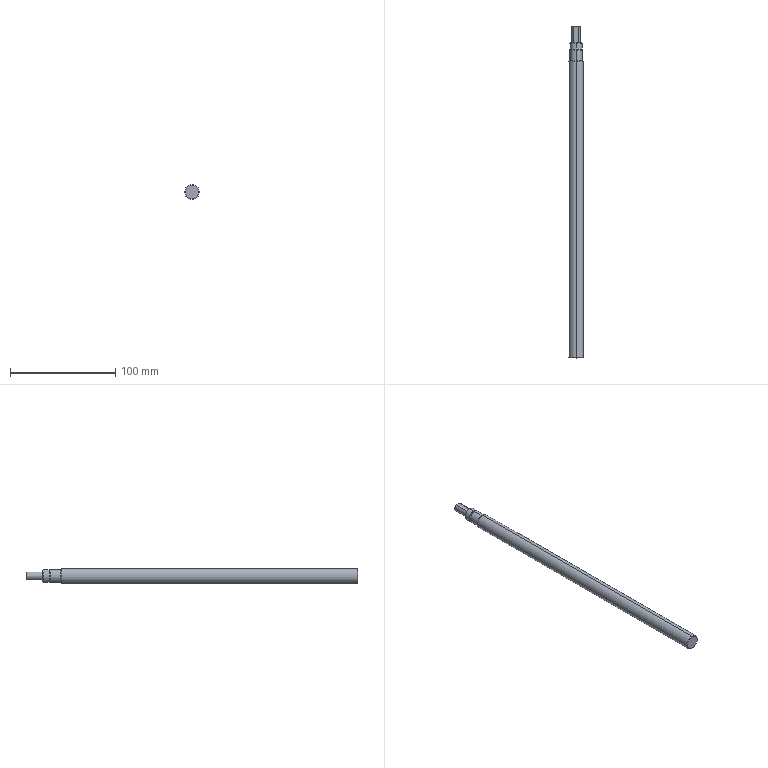Component | SolidWorks | CCDJSAdjustingScrew01-1 | 1 solid | 26 faces | box 14 x 315 x 14 mm | volume 46051 mm3 | cylinder 10 | cone 8 | plane 8 | commonest cylinder face diameters 12 x4 11.3 x2 14 x2 8 x2
build123d program:
from build123d import *

# Parameters (mm, degrees)
SKETCH2_R           = 4
BOSS_EXTRUDE1_DEPTH = 16
CHAMFER1_SIZE       = 0.5
SKETCH3_R           = 6
SKETCH3_W           = 9
SKETCH3_H           = 6.8
CUT_EXTRUDE1_DEPTH  = 16
CUT_EXTRUDE2_START  = 10
SKETCH4_OUTSIDE_W   = 79.124
SKETCH4_OUTSIDE_H   = 79.124
SKETCH4_OUTSIDE_R   = 5.65
CUT_EXTRUDE2_DEPTH  = 1.1


with BuildPart() as part:
    # Sketch1 → Revolve1 (revolve)
    with BuildSketch(Plane.XY, mode=Mode.PRIVATE) as revolve1_sk:
        Polygon((0, 0), (7, 0), (7, 282), (6, 282), (6, 299), (0, 299), align=None)
    revolve(revolve1_sk.sketch.rotate(Axis((0, 0, 0), (0, 1, 0)), 90), axis=Axis((0, 0, 0), (0, 1, 0)))

    # Sketch2 → Boss-Extrude1 (add)
    with BuildSketch(Plane(origin=(0, 299, 0), x_dir=(1, 0, 0), z_dir=(0, 1, 0))):
        with Locations(Location((0, 0, 0), (0, 0, 270))):
            Circle(SKETCH2_R)
    extrude(amount=BOSS_EXTRUDE1_DEPTH)

    # Chamfer1
    chamfer1_edges = [part.edges().sort_by_distance(p)[0] for p in [
        (0, 315, -4),
        (0, 299, 6),
        (0, 282, 7),
        (0, 0, 7),
    ]]
    chamfer(chamfer1_edges, length=CHAMFER1_SIZE)

    # Sketch3 → Cut-Extrude1 (cut)
    with BuildSketch(Plane(origin=(0, 315, 0), x_dir=(1, 0, 0), z_dir=(0, 1, 0))):
        with Locations(Location((0, 0, 0), (0, 0, 90))):
            Circle(SKETCH3_R)
        Rectangle(SKETCH3_W, SKETCH3_H, mode=Mode.SUBTRACT)
    extrude(amount=-CUT_EXTRUDE1_DEPTH, mode=Mode.SUBTRACT)

    # Sketch4 outside → Cut-Extrude2 (cut)
    with BuildSketch(Plane(origin=(0, 282, 0), x_dir=(1, 0, 0), z_dir=(0, 1, 0)).offset(CUT_EXTRUDE2_START)):
        Rectangle(SKETCH4_OUTSIDE_W, SKETCH4_OUTSIDE_H)
        with Locations(Location((0, 0, 0), (0, 0, 270))):
            Circle(SKETCH4_OUTSIDE_R, mode=Mode.SUBTRACT)
    extrude(amount=CUT_EXTRUDE2_DEPTH, mode=Mode.SUBTRACT)


solid = part.part

# Placed as in the assembly
solid = solid.moved(Location((0, 244.564, 0), (0, 0, 0)))
STEP:
#1=COLOUR_RGB('',0.7922,0.8196,0.9333);
#2=FILL_AREA_STYLE_COLOUR('',#1);
#3=FILL_AREA_STYLE('',(#2));
#4=SURFACE_STYLE_FILL_AREA(#3);
#5=SURFACE_SIDE_STYLE('',(#4));
#6=SURFACE_STYLE_USAGE(.BOTH.,#5);
#7=PRESENTATION_STYLE_ASSIGNMENT((#6));
#8=CARTESIAN_POINT('',(-0.,21.38,-0.2362));
#9=VERTEX_POINT('',#8);
#10=CARTESIAN_POINT('',(-0.,21.38,0.2362));
#11=VERTEX_POINT('',#10);
#12=CARTESIAN_POINT('',(-0.,21.38,-0.));
#13=DIRECTION('',(0.,-1.,0.));
#14=DIRECTION('',(0.,0.,1.));
#15=AXIS2_PLACEMENT_3D('',#12,#13,#14);
#16=CIRCLE('',#15,0.2362);
#17=EDGE_CURVE('',#9,#11,#16,.T.);
#18=ORIENTED_EDGE('',*,*,#17,.T.);
#19=CARTESIAN_POINT('',(-0.,21.168,0.2362));
#20=VERTEX_POINT('',#19);
#21=CARTESIAN_POINT('',(-0.,9.629,0.2362));
#22=DIRECTION('',(0.,-1.,0.));
#23=VECTOR('',#22,39.37);
#24=LINE('',#21,#23);
#25=EDGE_CURVE('',#11,#20,#24,.T.);
#26=ORIENTED_EDGE('',*,*,#25,.T.);
#27=CARTESIAN_POINT('',(-0.,21.168,-0.2362));
#28=VERTEX_POINT('',#27);
#29=CARTESIAN_POINT('',(-0.,21.168,-0.));
#30=DIRECTION('',(0.,-1.,0.));
#31=DIRECTION('',(0.,0.,1.));
#32=AXIS2_PLACEMENT_3D('',#29,#30,#31);
#33=CIRCLE('',#32,0.2362);
#34=EDGE_CURVE('',#28,#20,#33,.T.);
#35=ORIENTED_EDGE('',*,*,#34,.F.);
#36=CARTESIAN_POINT('',(-0.,9.629,-0.2362));
#37=DIRECTION('',(0.,-1.,0.));
#38=VECTOR('',#37,39.37);
#39=LINE('',#36,#38);
#40=EDGE_CURVE('',#9,#28,#39,.T.);
#41=ORIENTED_EDGE('',*,*,#40,.F.);
#42=EDGE_LOOP('',(#18,#26,#35,#41));
#43=FACE_OUTER_BOUND('',#42,.T.);
#44=CARTESIAN_POINT('',(-0.,9.629,-0.));
#45=DIRECTION('',(0.,-1.,0.));
#46=DIRECTION('',(0.,0.,-1.));
#47=AXIS2_PLACEMENT_3D('',#44,#45,#46);
#48=CYLINDRICAL_SURFACE('',#47,0.2362);
#49=ADVANCED_FACE('',(#43),#48,.T.);
#50=CARTESIAN_POINT('',(-0.,21.4,0.2165));
#51=VERTEX_POINT('',#50);
#52=CARTESIAN_POINT('',(-0.,21.4,-0.2165));
#53=VERTEX_POINT('',#52);
#54=CARTESIAN_POINT('',(-0.,21.4,-0.));
#55=DIRECTION('',(0.,1.,0.));
#56=DIRECTION('',(0.,0.,1.));
#57=AXIS2_PLACEMENT_3D('',#54,#55,#56);
#58=CIRCLE('',#57,0.2165);
#59=EDGE_CURVE('',#51,#53,#58,.T.);
#60=ORIENTED_EDGE('',*,*,#59,.F.);
#61=CARTESIAN_POINT('',(-0.,21.38,0.2362));
#62=DIRECTION('',(0.,-0.7071,0.7071));
#63=VECTOR('',#62,39.37);
#64=LINE('',#61,#63);
#65=EDGE_CURVE('',#51,#11,#64,.T.);
#66=ORIENTED_EDGE('',*,*,#65,.T.);
#67=ORIENTED_EDGE('',*,*,#17,.F.);
#68=CARTESIAN_POINT('',(-0.,21.38,-0.2362));
#69=DIRECTION('',(0.,-0.7071,-0.7071));
#70=VECTOR('',#69,39.37);
#71=LINE('',#68,#70);
#72=EDGE_CURVE('',#53,#9,#71,.T.);
#73=ORIENTED_EDGE('',*,*,#72,.F.);
#74=EDGE_LOOP('',(#60,#66,#67,#73));
#75=FACE_OUTER_BOUND('',#74,.T.);
#76=CARTESIAN_POINT('',(-0.,21.38,-0.));
#77=DIRECTION('',(0.,-1.,0.));
#78=DIRECTION('',(0.,0.,-1.));
#79=AXIS2_PLACEMENT_3D('',#76,#77,#78);
#80=CONICAL_SURFACE('',#79,0.2362,0.7854);
#81=ADVANCED_FACE('',(#75),#80,.T.);
#82=CARTESIAN_POINT('',(-0.,21.168,0.2224));
#83=VERTEX_POINT('',#82);
#84=CARTESIAN_POINT('',(-0.,21.168,-0.2224));
#85=VERTEX_POINT('',#84);
#86=CARTESIAN_POINT('',(-0.,21.168,-0.));
#87=DIRECTION('',(0.,1.,0.));
#88=DIRECTION('',(0.,0.,1.));
#89=AXIS2_PLACEMENT_3D('',#86,#87,#88);
#90=CIRCLE('',#89,0.2224);
#91=EDGE_CURVE('',#83,#85,#90,.T.);
#92=ORIENTED_EDGE('',*,*,#91,.F.);
#93=CARTESIAN_POINT('',(-0.,21.125,0.2224));
#94=VERTEX_POINT('',#93);
#95=CARTESIAN_POINT('',(-0.,21.168,0.2224));
#96=DIRECTION('',(0.,-1.,0.));
#97=VECTOR('',#96,39.37);
#98=LINE('',#95,#97);
#99=EDGE_CURVE('',#83,#94,#98,.T.);
#100=ORIENTED_EDGE('',*,*,#99,.T.);
#101=CARTESIAN_POINT('',(-0.,21.125,-0.2224));
#102=VERTEX_POINT('',#101);
#103=CARTESIAN_POINT('',(-0.,21.125,-0.));
#104=DIRECTION('',(0.,1.,0.));
#105=DIRECTION('',(0.,0.,1.));
#106=AXIS2_PLACEMENT_3D('',#103,#104,#105);
#107=CIRCLE('',#106,0.2224);
#108=EDGE_CURVE('',#94,#102,#107,.T.);
#109=ORIENTED_EDGE('',*,*,#108,.T.);
#110=CARTESIAN_POINT('',(-0.,21.168,-0.2224));
#111=DIRECTION('',(0.,-1.,0.));
#112=VECTOR('',#111,39.37);
#113=LINE('',#110,#112);
#114=EDGE_CURVE('',#85,#102,#113,.T.);
#115=ORIENTED_EDGE('',*,*,#114,.F.);
#116=EDGE_LOOP('',(#92,#100,#109,#115));
#117=FACE_OUTER_BOUND('',#116,.T.);
#118=CARTESIAN_POINT('',(-0.,21.168,-0.));
#119=DIRECTION('',(0.,-1.,0.));
#120=DIRECTION('',(0.,0.,-1.));
#121=AXIS2_PLACEMENT_3D('',#118,#119,#120);
#122=CYLINDRICAL_SURFACE('',#121,0.2224);
#123=ADVANCED_FACE('',(#117),#122,.T.);
#124=CARTESIAN_POINT('',(-0.,20.731,0.2559));
#125=VERTEX_POINT('',#124);
#126=CARTESIAN_POINT('',(-0.,20.731,-0.2559));
#127=VERTEX_POINT('',#126);
#128=CARTESIAN_POINT('',(-0.,20.731,-0.));
#129=DIRECTION('',(0.,1.,0.));
#130=DIRECTION('',(0.,0.,1.));
#131=AXIS2_PLACEMENT_3D('',#128,#129,#130);
#132=CIRCLE('',#131,0.2559);
#133=EDGE_CURVE('',#125,#127,#132,.T.);
#134=ORIENTED_EDGE('',*,*,#133,.F.);
#135=CARTESIAN_POINT('',(-0.,20.711,0.2756));
#136=VERTEX_POINT('',#135);
#137=CARTESIAN_POINT('',(-0.,20.711,0.2756));
#138=DIRECTION('',(0.,-0.7071,0.7071));
#139=VECTOR('',#138,39.37);
#140=LINE('',#137,#139);
#141=EDGE_CURVE('',#125,#136,#140,.T.);
#142=ORIENTED_EDGE('',*,*,#141,.T.);
#143=CARTESIAN_POINT('',(-0.,20.711,-0.2756));
#144=VERTEX_POINT('',#143);
#145=CARTESIAN_POINT('',(-0.,20.711,-0.));
#146=DIRECTION('',(0.,-1.,0.));
#147=DIRECTION('',(0.,0.,1.));
#148=AXIS2_PLACEMENT_3D('',#145,#146,#147);
#149=CIRCLE('',#148,0.2756);
#150=EDGE_CURVE('',#144,#136,#149,.T.);
#151=ORIENTED_EDGE('',*,*,#150,.F.);
#152=CARTESIAN_POINT('',(-0.,20.711,-0.2756));
#153=DIRECTION('',(0.,-0.7071,-0.7071));
#154=VECTOR('',#153,39.37);
#155=LINE('',#152,#154);
#156=EDGE_CURVE('',#127,#144,#155,.T.);
#157=ORIENTED_EDGE('',*,*,#156,.F.);
#158=EDGE_LOOP('',(#134,#142,#151,#157));
#159=FACE_OUTER_BOUND('',#158,.T.);
#160=CARTESIAN_POINT('',(-0.,20.711,-0.));
#161=DIRECTION('',(0.,-1.,0.));
#162=DIRECTION('',(0.,0.,-1.));
#163=AXIS2_PLACEMENT_3D('',#160,#161,#162);
#164=CONICAL_SURFACE('',#163,0.2756,0.7854);
#165=ADVANCED_FACE('',(#159),#164,.T.);
#166=CARTESIAN_POINT('',(-0.,9.629,-0.2559));
#167=VERTEX_POINT('',#166);
#168=CARTESIAN_POINT('',(-0.,9.629,0.2559));
#169=VERTEX_POINT('',#168);
#170=CARTESIAN_POINT('',(-0.,9.629,-0.));
#171=DIRECTION('',(0.,-1.,0.));
#172=DIRECTION('',(0.,0.,-1.));
#173=AXIS2_PLACEMENT_3D('',#170,#171,#172);
#174=CIRCLE('',#173,0.2559);
#175=EDGE_CURVE('',#167,#169,#174,.T.);
#176=ORIENTED_EDGE('',*,*,#175,.F.);
#177=CARTESIAN_POINT('',(-0.,9.648,-0.2756));
#178=VERTEX_POINT('',#177);
#179=CARTESIAN_POINT('',(-0.,9.629,-0.2559));
#180=DIRECTION('',(0.,0.7071,-0.7071));
#181=VECTOR('',#180,39.37);
#182=LINE('',#179,#181);
#183=EDGE_CURVE('',#167,#178,#182,.T.);
#184=ORIENTED_EDGE('',*,*,#183,.T.);
#185=CARTESIAN_POINT('',(-0.,9.648,0.2756));
#186=VERTEX_POINT('',#185);
#187=CARTESIAN_POINT('',(-0.,9.648,-0.));
#188=DIRECTION('',(0.,1.,0.));
#189=DIRECTION('',(0.,0.,-1.));
#190=AXIS2_PLACEMENT_3D('',#187,#188,#189);
#191=CIRCLE('',#190,0.2756);
#192=EDGE_CURVE('',#186,#178,#191,.T.);
#193=ORIENTED_EDGE('',*,*,#192,.F.);
#194=CARTESIAN_POINT('',(-0.,9.629,0.2559));
#195=DIRECTION('',(0.,0.7071,0.7071));
#196=VECTOR('',#195,39.37);
#197=LINE('',#194,#196);
#198=EDGE_CURVE('',#169,#186,#197,.T.);
#199=ORIENTED_EDGE('',*,*,#198,.F.);
#200=EDGE_LOOP('',(#176,#184,#193,#199));
#201=FACE_OUTER_BOUND('',#200,.T.);
#202=CARTESIAN_POINT('',(-0.,9.629,-0.));
#203=DIRECTION('',(0.,1.,0.));
#204=DIRECTION('',(0.,0.,1.));
#205=AXIS2_PLACEMENT_3D('',#202,#203,#204);
#206=CONICAL_SURFACE('',#205,0.2559,0.7854);
#207=ADVANCED_FACE('',(#201),#206,.T.);
#208=ORIENTED_EDGE('',*,*,#150,.T.);
#209=CARTESIAN_POINT('',(-0.,9.629,0.2756));
#210=DIRECTION('',(0.,-1.,0.));
#211=VECTOR('',#210,39.37);
#212=LINE('',#209,#211);
#213=EDGE_CURVE('',#136,#186,#212,.T.);
#214=ORIENTED_EDGE('',*,*,#213,.T.);
#215=ORIENTED_EDGE('',*,*,#192,.T.);
#216=CARTESIAN_POINT('',(-0.,9.629,-0.2756));
#217=DIRECTION('',(0.,-1.,0.));
#218=VECTOR('',#217,39.37);
#219=LINE('',#216,#218);
#220=EDGE_CURVE('',#144,#178,#219,.T.);
#221=ORIENTED_EDGE('',*,*,#220,.F.);
#222=EDGE_LOOP('',(#208,#214,#215,#221));
#223=FACE_OUTER_BOUND('',#222,.T.);
#224=CARTESIAN_POINT('',(-0.,9.629,-0.));
#225=DIRECTION('',(0.,-1.,0.));
#226=DIRECTION('',(0.,0.,-1.));
#227=AXIS2_PLACEMENT_3D('',#224,#225,#226);
#228=CYLINDRICAL_SURFACE('',#227,0.2756);
#229=ADVANCED_FACE('',(#223),#228,.T.);
#230=CARTESIAN_POINT('',(-0.,21.125,-0.2362));
#231=VERTEX_POINT('',#230);
#232=CARTESIAN_POINT('',(-0.,21.125,0.2362));
#233=VERTEX_POINT('',#232);
#234=CARTESIAN_POINT('',(-0.,21.125,-0.));
#235=DIRECTION('',(0.,-1.,0.));
#236=DIRECTION('',(0.,0.,1.));
#237=AXIS2_PLACEMENT_3D('',#234,#235,#236);
#238=CIRCLE('',#237,0.2362);
#239=EDGE_CURVE('',#231,#233,#238,.T.);
#240=ORIENTED_EDGE('',*,*,#239,.T.);
#241=CARTESIAN_POINT('',(-0.,20.731,0.2362));
#242=VERTEX_POINT('',#241);
#243=CARTESIAN_POINT('',(-0.,9.629,0.2362));
#244=DIRECTION('',(0.,-1.,0.));
#245=VECTOR('',#244,39.37);
#246=LINE('',#243,#245);
#247=EDGE_CURVE('',#233,#242,#246,.T.);
#248=ORIENTED_EDGE('',*,*,#247,.T.);
#249=CARTESIAN_POINT('',(-0.,20.731,-0.2362));
#250=VERTEX_POINT('',#249);
#251=CARTESIAN_POINT('',(-0.,20.731,-0.));
#252=DIRECTION('',(0.,-1.,0.));
#253=DIRECTION('',(0.,0.,-1.));
#254=AXIS2_PLACEMENT_3D('',#251,#252,#253);
#255=CIRCLE('',#254,0.2362);
#256=EDGE_CURVE('',#250,#242,#255,.T.);
#257=ORIENTED_EDGE('',*,*,#256,.F.);
#258=CARTESIAN_POINT('',(-0.,9.629,-0.2362));
#259=DIRECTION('',(0.,-1.,0.));
#260=VECTOR('',#259,39.37);
#261=LINE('',#258,#260);
#262=EDGE_CURVE('',#231,#250,#261,.T.);
#263=ORIENTED_EDGE('',*,*,#262,.F.);
#264=EDGE_LOOP('',(#240,#248,#257,#263));
#265=FACE_OUTER_BOUND('',#264,.T.);
#266=CARTESIAN_POINT('',(-0.,9.629,-0.));
#267=DIRECTION('',(0.,-1.,0.));
#268=DIRECTION('',(0.,0.,-1.));
#269=AXIS2_PLACEMENT_3D('',#266,#267,#268);
#270=CYLINDRICAL_SURFACE('',#269,0.2362);
#271=ADVANCED_FACE('',(#265),#270,.T.);
#272=ORIENTED_EDGE('',*,*,#247,.F.);
#273=CARTESIAN_POINT('',(-0.,21.125,-0.));
#274=DIRECTION('',(0.,-1.,0.));
#275=DIRECTION('',(0.,0.,1.));
#276=AXIS2_PLACEMENT_3D('',#273,#274,#275);
#277=CIRCLE('',#276,0.2362);
#278=EDGE_CURVE('',#233,#231,#277,.T.);
#279=ORIENTED_EDGE('',*,*,#278,.T.);
#280=ORIENTED_EDGE('',*,*,#262,.T.);
#281=CARTESIAN_POINT('',(-0.,20.731,-0.));
#282=DIRECTION('',(0.,-1.,0.));
#283=DIRECTION('',(0.,0.,-1.));
#284=AXIS2_PLACEMENT_3D('',#281,#282,#283);
#285=CIRCLE('',#284,0.2362);
#286=EDGE_CURVE('',#242,#250,#285,.T.);
#287=ORIENTED_EDGE('',*,*,#286,.F.);
#288=EDGE_LOOP('',(#272,#279,#280,#287));
#289=FACE_OUTER_BOUND('',#288,.T.);
#290=CARTESIAN_POINT('',(-0.,9.629,-0.));
#291=DIRECTION('',(0.,-1.,0.));
#292=DIRECTION('',(0.,0.,-1.));
#293=AXIS2_PLACEMENT_3D('',#290,#291,#292);
#294=CYLINDRICAL_SURFACE('',#293,0.2362);
#295=ADVANCED_FACE('',(#289),#294,.T.);
#296=CARTESIAN_POINT('',(-0.,9.629,-0.));
#297=DIRECTION('',(0.,-1.,0.));
#298=DIRECTION('',(0.,0.,-1.));
#299=AXIS2_PLACEMENT_3D('',#296,#297,#298);
#300=CIRCLE('',#299,0.2559);
#301=EDGE_CURVE('',#169,#167,#300,.T.);
#302=ORIENTED_EDGE('',*,*,#301,.T.);
#303=ORIENTED_EDGE('',*,*,#175,.T.);
#304=EDGE_LOOP('',(#302,#303));
#305=FACE_OUTER_BOUND('',#304,.T.);
#306=CARTESIAN_POINT('',(-0.,9.629,-0.));
#307=DIRECTION('',(0.,-1.,0.));
#308=DIRECTION('',(0.,0.,-1.));
#309=AXIS2_PLACEMENT_3D('',#306,#307,#308);
#310=PLANE('',#309);
#311=ADVANCED_FACE('',(#305),#310,.T.);
#312=ORIENTED_EDGE('',*,*,#213,.F.);
#313=CARTESIAN_POINT('',(-0.,20.711,-0.));
#314=DIRECTION('',(0.,-1.,0.));
#315=DIRECTION('',(0.,0.,1.));
#316=AXIS2_PLACEMENT_3D('',#313,#314,#315);
#317=CIRCLE('',#316,0.2756);
#318=EDGE_CURVE('',#136,#144,#317,.T.);
#319=ORIENTED_EDGE('',*,*,#318,.T.);
#320=ORIENTED_EDGE('',*,*,#220,.T.);
#321=CARTESIAN_POINT('',(-0.,9.648,-0.));
#322=DIRECTION('',(0.,1.,0.));
#323=DIRECTION('',(0.,0.,-1.));
#324=AXIS2_PLACEMENT_3D('',#321,#322,#323);
#325=CIRCLE('',#324,0.2756);
#326=EDGE_CURVE('',#178,#186,#325,.T.);
#327=ORIENTED_EDGE('',*,*,#326,.T.);
#328=EDGE_LOOP('',(#312,#319,#320,#327));
#329=FACE_OUTER_BOUND('',#328,.T.);
#330=CARTESIAN_POINT('',(-0.,9.629,-0.));
#331=DIRECTION('',(0.,-1.,0.));
#332=DIRECTION('',(0.,0.,-1.));
#333=AXIS2_PLACEMENT_3D('',#330,#331,#332);
#334=CYLINDRICAL_SURFACE('',#333,0.2756);
#335=ADVANCED_FACE('',(#329),#334,.T.);
#336=CARTESIAN_POINT('',(-0.,20.731,-0.));
#337=DIRECTION('',(0.,1.,0.));
#338=DIRECTION('',(0.,0.,1.));
#339=AXIS2_PLACEMENT_3D('',#336,#337,#338);
#340=CIRCLE('',#339,0.2559);
#341=EDGE_CURVE('',#127,#125,#340,.T.);
#342=ORIENTED_EDGE('',*,*,#341,.T.);
#343=ORIENTED_EDGE('',*,*,#133,.T.);
#344=EDGE_LOOP('',(#342,#343));
#345=FACE_OUTER_BOUND('',#344,.T.);
#346=ORIENTED_EDGE('',*,*,#256,.T.);
#347=ORIENTED_EDGE('',*,*,#286,.T.);
#348=EDGE_LOOP('',(#346,#347));
#349=FACE_BOUND('',#348,.T.);
#350=CARTESIAN_POINT('',(0.2756,20.731,-0.));
#351=DIRECTION('',(0.,1.,0.));
#352=DIRECTION('',(0.,0.,1.));
#353=AXIS2_PLACEMENT_3D('',#350,#351,#352);
#354=PLANE('',#353);
#355=ADVANCED_FACE('',(#345,#349),#354,.T.);
#356=ORIENTED_EDGE('',*,*,#183,.F.);
#357=ORIENTED_EDGE('',*,*,#301,.F.);
#358=ORIENTED_EDGE('',*,*,#198,.T.);
#359=ORIENTED_EDGE('',*,*,#326,.F.);
#360=EDGE_LOOP('',(#356,#357,#358,#359));
#361=FACE_OUTER_BOUND('',#360,.T.);
#362=CARTESIAN_POINT('',(-0.,9.629,-0.));
#363=DIRECTION('',(0.,1.,0.));
#364=DIRECTION('',(0.,0.,1.));
#365=AXIS2_PLACEMENT_3D('',#362,#363,#364);
#366=CONICAL_SURFACE('',#365,0.2559,0.7854);
#367=ADVANCED_FACE('',(#361),#366,.T.);
#368=ORIENTED_EDGE('',*,*,#141,.F.);
#369=ORIENTED_EDGE('',*,*,#341,.F.);
#370=ORIENTED_EDGE('',*,*,#156,.T.);
#371=ORIENTED_EDGE('',*,*,#318,.F.);
#372=EDGE_LOOP('',(#368,#369,#370,#371));
#373=FACE_OUTER_BOUND('',#372,.T.);
#374=CARTESIAN_POINT('',(-0.,20.711,-0.));
#375=DIRECTION('',(0.,-1.,0.));
#376=DIRECTION('',(0.,0.,-1.));
#377=AXIS2_PLACEMENT_3D('',#374,#375,#376);
#378=CONICAL_SURFACE('',#377,0.2756,0.7854);
#379=ADVANCED_FACE('',(#373),#378,.T.);
#380=ORIENTED_EDGE('',*,*,#34,.T.);
#381=CARTESIAN_POINT('',(-0.,21.168,-0.));
#382=DIRECTION('',(0.,-1.,0.));
#383=DIRECTION('',(0.,0.,1.));
#384=AXIS2_PLACEMENT_3D('',#381,#382,#383);
#385=CIRCLE('',#384,0.2362);
#386=EDGE_CURVE('',#20,#28,#385,.T.);
#387=ORIENTED_EDGE('',*,*,#386,.T.);
#388=EDGE_LOOP('',(#380,#387));
#389=FACE_OUTER_BOUND('',#388,.T.);
#390=CARTESIAN_POINT('',(-0.,21.168,-0.));
#391=DIRECTION('',(0.,1.,0.));
#392=DIRECTION('',(0.,0.,1.));
#393=AXIS2_PLACEMENT_3D('',#390,#391,#392);
#394=CIRCLE('',#393,0.2224);
#395=EDGE_CURVE('',#85,#83,#394,.T.);
#396=ORIENTED_EDGE('',*,*,#395,.T.);
#397=ORIENTED_EDGE('',*,*,#91,.T.);
#398=EDGE_LOOP('',(#396,#397));
#399=FACE_BOUND('',#398,.T.);
#400=CARTESIAN_POINT('',(-0.,21.168,-0.));
#401=DIRECTION('',(0.,1.,0.));
#402=DIRECTION('',(0.,0.,1.));
#403=AXIS2_PLACEMENT_3D('',#400,#401,#402);
#404=PLANE('',#403);
#405=ADVANCED_FACE('',(#389,#399),#404,.F.);
#406=ORIENTED_EDGE('',*,*,#239,.F.);
#407=ORIENTED_EDGE('',*,*,#278,.F.);
#408=EDGE_LOOP('',(#406,#407));
#409=FACE_OUTER_BOUND('',#408,.T.);
#410=CARTESIAN_POINT('',(-0.,21.125,-0.));
#411=DIRECTION('',(0.,1.,0.));
#412=DIRECTION('',(0.,0.,1.));
#413=AXIS2_PLACEMENT_3D('',#410,#411,#412);
#414=CIRCLE('',#413,0.2224);
#415=EDGE_CURVE('',#102,#94,#414,.T.);
#416=ORIENTED_EDGE('',*,*,#415,.F.);
#417=ORIENTED_EDGE('',*,*,#108,.F.);
#418=EDGE_LOOP('',(#416,#417));
#419=FACE_BOUND('',#418,.T.);
#420=CARTESIAN_POINT('',(-0.,21.125,-0.));
#421=DIRECTION('',(0.,1.,0.));
#422=DIRECTION('',(0.,0.,1.));
#423=AXIS2_PLACEMENT_3D('',#420,#421,#422);
#424=PLANE('',#423);
#425=ADVANCED_FACE('',(#409,#419),#424,.T.);
#426=ORIENTED_EDGE('',*,*,#99,.F.);
#427=ORIENTED_EDGE('',*,*,#395,.F.);
#428=ORIENTED_EDGE('',*,*,#114,.T.);
#429=ORIENTED_EDGE('',*,*,#415,.T.);
#430=EDGE_LOOP('',(#426,#427,#428,#429));
#431=FACE_OUTER_BOUND('',#430,.T.);
#432=CARTESIAN_POINT('',(-0.,21.168,-0.));
#433=DIRECTION('',(0.,-1.,0.));
#434=DIRECTION('',(0.,0.,-1.));
#435=AXIS2_PLACEMENT_3D('',#432,#433,#434);
#436=CYLINDRICAL_SURFACE('',#435,0.2224);
#437=ADVANCED_FACE('',(#431),#436,.T.);
#438=CARTESIAN_POINT('',(0.08296,22.01,-0.1339));
#439=VERTEX_POINT('',#438);
#440=CARTESIAN_POINT('',(0.08296,22.01,0.1339));
#441=VERTEX_POINT('',#440);
#442=CARTESIAN_POINT('',(-0.,22.01,-0.));
#443=DIRECTION('',(0.,-1.,0.));
#444=DIRECTION('',(-0.,0.,1.));
#445=AXIS2_PLACEMENT_3D('',#442,#443,#444);
#446=CIRCLE('',#445,0.1575);
#447=EDGE_CURVE('',#439,#441,#446,.T.);
#448=ORIENTED_EDGE('',*,*,#447,.F.);
#449=CARTESIAN_POINT('',(0.0327,22.03,-0.1339));
#450=VERTEX_POINT('',#449);
#451=CARTESIAN_POINT('',(0.08296,22.01,-0.1339));
#452=CARTESIAN_POINT('',(0.07499,22.015,-0.1339));
#453=CARTESIAN_POINT('',(0.06686,22.018,-0.1339));
#454=CARTESIAN_POINT('',(0.05012,22.025,-0.1339));
#455=CARTESIAN_POINT('',(0.04146,22.028,-0.1339));
#456=CARTESIAN_POINT('',(0.0327,22.03,-0.1339));
#457=B_SPLINE_CURVE_WITH_KNOTS('',3,(#451,#452,#453,#454,#455,#456),.UNSPECIFIED.,.F.,.F.,(4,2,4),(0.007723,0.00841,0.009097),.UNSPECIFIED.);
#458=EDGE_CURVE('',#439,#450,#457,.T.);
#459=ORIENTED_EDGE('',*,*,#458,.T.);
#460=CARTESIAN_POINT('',(0.0327,22.03,0.1339));
#461=VERTEX_POINT('',#460);
#462=CARTESIAN_POINT('',(-0.,22.03,-0.));
#463=DIRECTION('',(0.,1.,0.));
#464=DIRECTION('',(0.,0.,1.));
#465=AXIS2_PLACEMENT_3D('',#462,#463,#464);
#466=CIRCLE('',#465,0.1378);
#467=EDGE_CURVE('',#461,#450,#466,.T.);
#468=ORIENTED_EDGE('',*,*,#467,.F.);
#469=CARTESIAN_POINT('',(0.0327,22.03,0.1339));
#470=CARTESIAN_POINT('',(0.04147,22.028,0.1339));
#471=CARTESIAN_POINT('',(0.05015,22.025,0.1339));
#472=CARTESIAN_POINT('',(0.06693,22.018,0.1339));
#473=CARTESIAN_POINT('',(0.07504,22.015,0.1339));
#474=CARTESIAN_POINT('',(0.08296,22.01,0.1339));
#475=B_SPLINE_CURVE_WITH_KNOTS('',3,(#469,#470,#471,#472,#473,#474),.UNSPECIFIED.,.F.,.F.,(4,2,4),(0.01078,0.01147,0.01215),.UNSPECIFIED.);
#476=EDGE_CURVE('',#461,#441,#475,.T.);
#477=ORIENTED_EDGE('',*,*,#476,.T.);
#478=EDGE_LOOP('',(#448,#459,#468,#477));
#479=FACE_OUTER_BOUND('',#478,.T.);
#480=CARTESIAN_POINT('',(-0.,22.03,-0.));
#481=DIRECTION('',(0.,-1.,0.));
#482=DIRECTION('',(0.,0.,-1.));
#483=AXIS2_PLACEMENT_3D('',#480,#481,#482);
#484=CONICAL_SURFACE('',#483,0.1378,0.7854);
#485=ADVANCED_FACE('',(#479),#484,.T.);
#486=ORIENTED_EDGE('',*,*,#467,.T.);
#487=CARTESIAN_POINT('',(-0.0327,22.03,-0.1339));
#488=VERTEX_POINT('',#487);
#489=CARTESIAN_POINT('',(-0.1772,22.03,-0.1339));
#490=DIRECTION('',(-1.,0.,0.));
#491=VECTOR('',#490,39.37);
#492=LINE('',#489,#491);
#493=EDGE_CURVE('',#450,#488,#492,.T.);
#494=ORIENTED_EDGE('',*,*,#493,.T.);
#495=CARTESIAN_POINT('',(-0.0327,22.03,0.1339));
#496=VERTEX_POINT('',#495);
#497=CARTESIAN_POINT('',(-0.,22.03,-0.));
#498=DIRECTION('',(0.,1.,0.));
#499=DIRECTION('',(0.,0.,1.));
#500=AXIS2_PLACEMENT_3D('',#497,#498,#499);
#501=CIRCLE('',#500,0.1378);
#502=EDGE_CURVE('',#488,#496,#501,.T.);
#503=ORIENTED_EDGE('',*,*,#502,.T.);
#504=CARTESIAN_POINT('',(-0.1772,22.03,0.1339));
#505=DIRECTION('',(1.,0.,0.));
#506=VECTOR('',#505,39.37);
#507=LINE('',#504,#506);
#508=EDGE_CURVE('',#496,#461,#507,.T.);
#509=ORIENTED_EDGE('',*,*,#508,.T.);
#510=EDGE_LOOP('',(#486,#494,#503,#509));
#511=FACE_OUTER_BOUND('',#510,.T.);
#512=CARTESIAN_POINT('',(-0.,22.03,-0.));
#513=DIRECTION('',(0.,1.,0.));
#514=DIRECTION('',(0.,0.,1.));
#515=AXIS2_PLACEMENT_3D('',#512,#513,#514);
#516=PLANE('',#515);
#517=ADVANCED_FACE('',(#511),#516,.T.);
#518=ORIENTED_EDGE('',*,*,#502,.F.);
#519=CARTESIAN_POINT('',(-0.08296,22.01,-0.1339));
#520=VERTEX_POINT('',#519);
#521=CARTESIAN_POINT('',(-0.0327,22.03,-0.1339));
#522=CARTESIAN_POINT('',(-0.04147,22.028,-0.1339));
#523=CARTESIAN_POINT('',(-0.05015,22.025,-0.1339));
#524=CARTESIAN_POINT('',(-0.06693,22.018,-0.1339));
#525=CARTESIAN_POINT('',(-0.07504,22.015,-0.1339));
#526=CARTESIAN_POINT('',(-0.08296,22.01,-0.1339));
#527=B_SPLINE_CURVE_WITH_KNOTS('',3,(#521,#522,#523,#524,#525,#526),.UNSPECIFIED.,.F.,.F.,(4,2,4),(0.01078,0.01147,0.01215),.UNSPECIFIED.);
#528=EDGE_CURVE('',#488,#520,#527,.T.);
#529=ORIENTED_EDGE('',*,*,#528,.T.);
#530=CARTESIAN_POINT('',(-0.08296,22.01,0.1339));
#531=VERTEX_POINT('',#530);
#532=CARTESIAN_POINT('',(-0.,22.01,-0.));
#533=DIRECTION('',(0.,-1.,0.));
#534=DIRECTION('',(0.,0.,1.));
#535=AXIS2_PLACEMENT_3D('',#532,#533,#534);
#536=CIRCLE('',#535,0.1575);
#537=EDGE_CURVE('',#531,#520,#536,.T.);
#538=ORIENTED_EDGE('',*,*,#537,.F.);
#539=CARTESIAN_POINT('',(-0.08296,22.01,0.1339));
#540=CARTESIAN_POINT('',(-0.07499,22.015,0.1339));
#541=CARTESIAN_POINT('',(-0.06686,22.018,0.1339));
#542=CARTESIAN_POINT('',(-0.05012,22.025,0.1339));
#543=CARTESIAN_POINT('',(-0.04146,22.028,0.1339));
#544=CARTESIAN_POINT('',(-0.0327,22.03,0.1339));
#545=B_SPLINE_CURVE_WITH_KNOTS('',3,(#539,#540,#541,#542,#543,#544),.UNSPECIFIED.,.F.,.F.,(4,2,4),(0.007723,0.00841,0.009097),.UNSPECIFIED.);
#546=EDGE_CURVE('',#531,#496,#545,.T.);
#547=ORIENTED_EDGE('',*,*,#546,.T.);
#548=EDGE_LOOP('',(#518,#529,#538,#547));
#549=FACE_OUTER_BOUND('',#548,.T.);
#550=CARTESIAN_POINT('',(-0.,22.03,-0.));
#551=DIRECTION('',(0.,-1.,0.));
#552=DIRECTION('',(0.,0.,-1.));
#553=AXIS2_PLACEMENT_3D('',#550,#551,#552);
#554=CONICAL_SURFACE('',#553,0.1378,0.7854);
#555=ADVANCED_FACE('',(#549),#554,.T.);
#556=CARTESIAN_POINT('',(-0.08296,21.4,-0.1339));
#557=VERTEX_POINT('',#556);
#558=CARTESIAN_POINT('',(-0.08296,22.03,-0.1339));
#559=DIRECTION('',(0.,1.,0.));
#560=VECTOR('',#559,39.37);
#561=LINE('',#558,#560);
#562=EDGE_CURVE('',#557,#520,#561,.T.);
#563=ORIENTED_EDGE('',*,*,#562,.F.);
#564=CARTESIAN_POINT('',(-0.08296,21.4,0.1339));
#565=VERTEX_POINT('',#564);
#566=CARTESIAN_POINT('',(-0.,21.4,-0.));
#567=DIRECTION('',(0.,1.,0.));
#568=DIRECTION('',(0.,0.,1.));
#569=AXIS2_PLACEMENT_3D('',#566,#567,#568);
#570=CIRCLE('',#569,0.1575);
#571=EDGE_CURVE('',#557,#565,#570,.T.);
#572=ORIENTED_EDGE('',*,*,#571,.T.);
#573=CARTESIAN_POINT('',(-0.08296,22.03,0.1339));
#574=DIRECTION('',(0.,-1.,0.));
#575=VECTOR('',#574,39.37);
#576=LINE('',#573,#575);
#577=EDGE_CURVE('',#531,#565,#576,.T.);
#578=ORIENTED_EDGE('',*,*,#577,.F.);
#579=ORIENTED_EDGE('',*,*,#537,.T.);
#580=EDGE_LOOP('',(#563,#572,#578,#579));
#581=FACE_OUTER_BOUND('',#580,.T.);
#582=CARTESIAN_POINT('',(-0.,22.03,-0.));
#583=DIRECTION('',(0.,-1.,0.));
#584=DIRECTION('',(0.,0.,-1.));
#585=AXIS2_PLACEMENT_3D('',#582,#583,#584);
#586=CYLINDRICAL_SURFACE('',#585,0.1575);
#587=ADVANCED_FACE('',(#581),#586,.T.);
#588=ORIENTED_EDGE('',*,*,#577,.T.);
#589=CARTESIAN_POINT('',(0.08296,21.4,0.1339));
#590=VERTEX_POINT('',#589);
#591=CARTESIAN_POINT('',(-0.1772,21.4,0.1339));
#592=DIRECTION('',(-1.,0.,0.));
#593=VECTOR('',#592,39.37);
#594=LINE('',#591,#593);
#595=EDGE_CURVE('',#590,#565,#594,.T.);
#596=ORIENTED_EDGE('',*,*,#595,.F.);
#597=CARTESIAN_POINT('',(0.08296,22.03,0.1339));
#598=DIRECTION('',(0.,1.,0.));
#599=VECTOR('',#598,39.37);
#600=LINE('',#597,#599);
#601=EDGE_CURVE('',#590,#441,#600,.T.);
#602=ORIENTED_EDGE('',*,*,#601,.T.);
#603=ORIENTED_EDGE('',*,*,#476,.F.);
#604=ORIENTED_EDGE('',*,*,#508,.F.);
#605=ORIENTED_EDGE('',*,*,#546,.F.);
#606=EDGE_LOOP('',(#588,#596,#602,#603,#604,#605));
#607=FACE_OUTER_BOUND('',#606,.T.);
#608=CARTESIAN_POINT('',(-0.1772,20.732,0.1339));
#609=DIRECTION('',(0.,0.,1.));
#610=DIRECTION('',(1.,0.,0.));
#611=AXIS2_PLACEMENT_3D('',#608,#609,#610);
#612=PLANE('',#611);
#613=ADVANCED_FACE('',(#607),#612,.T.);
#614=CARTESIAN_POINT('',(0.08296,21.4,-0.1339));
#615=VERTEX_POINT('',#614);
#616=CARTESIAN_POINT('',(0.08296,22.03,-0.1339));
#617=DIRECTION('',(0.,-1.,0.));
#618=VECTOR('',#617,39.37);
#619=LINE('',#616,#618);
#620=EDGE_CURVE('',#439,#615,#619,.T.);
#621=ORIENTED_EDGE('',*,*,#620,.F.);
#622=ORIENTED_EDGE('',*,*,#447,.T.);
#623=ORIENTED_EDGE('',*,*,#601,.F.);
#624=CARTESIAN_POINT('',(-0.,21.4,-0.));
#625=DIRECTION('',(0.,1.,0.));
#626=DIRECTION('',(0.,0.,1.));
#627=AXIS2_PLACEMENT_3D('',#624,#625,#626);
#628=CIRCLE('',#627,0.1575);
#629=EDGE_CURVE('',#590,#615,#628,.T.);
#630=ORIENTED_EDGE('',*,*,#629,.T.);
#631=EDGE_LOOP('',(#621,#622,#623,#630));
#632=FACE_OUTER_BOUND('',#631,.T.);
#633=CARTESIAN_POINT('',(-0.,22.03,-0.));
#634=DIRECTION('',(0.,-1.,0.));
#635=DIRECTION('',(0.,0.,-1.));
#636=AXIS2_PLACEMENT_3D('',#633,#634,#635);
#637=CYLINDRICAL_SURFACE('',#636,0.1575);
#638=ADVANCED_FACE('',(#632),#637,.T.);
#639=ORIENTED_EDGE('',*,*,#620,.T.);
#640=CARTESIAN_POINT('',(-0.1772,21.4,-0.1339));
#641=DIRECTION('',(1.,0.,0.));
#642=VECTOR('',#641,39.37);
#643=LINE('',#640,#642);
#644=EDGE_CURVE('',#557,#615,#643,.T.);
#645=ORIENTED_EDGE('',*,*,#644,.F.);
#646=ORIENTED_EDGE('',*,*,#562,.T.);
#647=ORIENTED_EDGE('',*,*,#528,.F.);
#648=ORIENTED_EDGE('',*,*,#493,.F.);
#649=ORIENTED_EDGE('',*,*,#458,.F.);
#650=EDGE_LOOP('',(#639,#645,#646,#647,#648,#649));
#651=FACE_OUTER_BOUND('',#650,.T.);
#652=CARTESIAN_POINT('',(-0.1772,20.732,-0.1339));
#653=DIRECTION('',(0.,0.,-1.));
#654=DIRECTION('',(-1.,0.,0.));
#655=AXIS2_PLACEMENT_3D('',#652,#653,#654);
#656=PLANE('',#655);
#657=ADVANCED_FACE('',(#651),#656,.T.);
#658=ORIENTED_EDGE('',*,*,#644,.T.);
#659=ORIENTED_EDGE('',*,*,#629,.F.);
#660=ORIENTED_EDGE('',*,*,#595,.T.);
#661=ORIENTED_EDGE('',*,*,#571,.F.);
#662=EDGE_LOOP('',(#658,#659,#660,#661));
#663=FACE_BOUND('',#662,.T.);
#664=CARTESIAN_POINT('',(-0.,21.4,-0.));
#665=DIRECTION('',(0.,1.,0.));
#666=DIRECTION('',(0.,0.,1.));
#667=AXIS2_PLACEMENT_3D('',#664,#665,#666);
#668=CIRCLE('',#667,0.2165);
#669=EDGE_CURVE('',#53,#51,#668,.T.);
#670=ORIENTED_EDGE('',*,*,#669,.T.);
#671=ORIENTED_EDGE('',*,*,#59,.T.);
#672=EDGE_LOOP('',(#670,#671));
#673=FACE_OUTER_BOUND('',#672,.T.);
#674=CARTESIAN_POINT('',(0.2362,21.4,-0.));
#675=DIRECTION('',(0.,1.,0.));
#676=DIRECTION('',(0.,0.,1.));
#677=AXIS2_PLACEMENT_3D('',#674,#675,#676);
#678=PLANE('',#677);
#679=ADVANCED_FACE('',(#663,#673),#678,.T.);
#680=ORIENTED_EDGE('',*,*,#65,.F.);
#681=ORIENTED_EDGE('',*,*,#669,.F.);
#682=ORIENTED_EDGE('',*,*,#72,.T.);
#683=CARTESIAN_POINT('',(-0.,21.38,-0.));
#684=DIRECTION('',(0.,-1.,0.));
#685=DIRECTION('',(0.,0.,1.));
#686=AXIS2_PLACEMENT_3D('',#683,#684,#685);
#687=CIRCLE('',#686,0.2362);
#688=EDGE_CURVE('',#11,#9,#687,.T.);
#689=ORIENTED_EDGE('',*,*,#688,.F.);
#690=EDGE_LOOP('',(#680,#681,#682,#689));
#691=FACE_OUTER_BOUND('',#690,.T.);
#692=CARTESIAN_POINT('',(-0.,21.38,-0.));
#693=DIRECTION('',(0.,-1.,0.));
#694=DIRECTION('',(0.,0.,-1.));
#695=AXIS2_PLACEMENT_3D('',#692,#693,#694);
#696=CONICAL_SURFACE('',#695,0.2362,0.7854);
#697=ADVANCED_FACE('',(#691),#696,.T.);
#698=ORIENTED_EDGE('',*,*,#25,.F.);
#699=ORIENTED_EDGE('',*,*,#688,.T.);
#700=ORIENTED_EDGE('',*,*,#40,.T.);
#701=ORIENTED_EDGE('',*,*,#386,.F.);
#702=EDGE_LOOP('',(#698,#699,#700,#701));
#703=FACE_OUTER_BOUND('',#702,.T.);
#704=CARTESIAN_POINT('',(-0.,9.629,-0.));
#705=DIRECTION('',(0.,-1.,0.));
#706=DIRECTION('',(0.,0.,-1.));
#707=AXIS2_PLACEMENT_3D('',#704,#705,#706);
#708=CYLINDRICAL_SURFACE('',#707,0.2362);
#709=ADVANCED_FACE('',(#703),#708,.T.);
#710=CLOSED_SHELL('',(#49,#81,#123,#165,#207,#229,#271,#295,#311,#335,#355,#367,#379,#405,#425,#437,#485,#517,#555,#587,#613,#638,#657,#679,#697,#709));
#711=MANIFOLD_SOLID_BREP('',#710);
#712=STYLED_ITEM('',(#7),#711);
#713=PRESENTATION_LAYER_ASSIGNMENT('','',(#712));
#714=CARTESIAN_POINT('',(0.,0.,0.));
#715=DIRECTION('',(0.,0.,1.));
#716=DIRECTION('',(1.,0.,0.));
#717=AXIS2_PLACEMENT_3D('',#714,#715,#716);
#718=(LENGTH_UNIT()NAMED_UNIT(*)SI_UNIT($,.METRE.));
#719=LENGTH_MEASURE_WITH_UNIT(LENGTH_MEASURE(0.0254),#718);
#720=DIMENSIONAL_EXPONENTS(1.,0.,0.,0.,0.,0.,0.);
#721=(CONVERSION_BASED_UNIT('',#719)LENGTH_UNIT()NAMED_UNIT(#720));
#722=UNCERTAINTY_MEASURE_WITH_UNIT(LENGTH_MEASURE(0.00001),#721,'','');
#723=(NAMED_UNIT(*)PLANE_ANGLE_UNIT()SI_UNIT($,.RADIAN.));
#724=(NAMED_UNIT(*)SI_UNIT($,.STERADIAN.)SOLID_ANGLE_UNIT());
#725=(GEOMETRIC_REPRESENTATION_CONTEXT(3)GLOBAL_UNCERTAINTY_ASSIGNED_CONTEXT((#722))GLOBAL_UNIT_ASSIGNED_CONTEXT((#721,#723,#724))REPRESENTATION_CONTEXT('',''));
#726=ADVANCED_BREP_SHAPE_REPRESENTATION('',(#711,#717),#725);
#727=(LENGTH_UNIT()NAMED_UNIT(*)SI_UNIT($,.METRE.));
#728=LENGTH_MEASURE_WITH_UNIT(LENGTH_MEASURE(0.0254),#727);
#729=DIMENSIONAL_EXPONENTS(1.,0.,0.,0.,0.,0.,0.);
#730=(CONVERSION_BASED_UNIT('',#728)LENGTH_UNIT()NAMED_UNIT(#729));
#731=UNCERTAINTY_MEASURE_WITH_UNIT(LENGTH_MEASURE(0.00001),#730,'','');
#732=(NAMED_UNIT(*)PLANE_ANGLE_UNIT()SI_UNIT($,.RADIAN.));
#733=(NAMED_UNIT(*)SI_UNIT($,.STERADIAN.)SOLID_ANGLE_UNIT());
#734=(GEOMETRIC_REPRESENTATION_CONTEXT(3)GLOBAL_UNCERTAINTY_ASSIGNED_CONTEXT((#731))GLOBAL_UNIT_ASSIGNED_CONTEXT((#730,#732,#733))REPRESENTATION_CONTEXT('',''));
#735=MECHANICAL_DESIGN_GEOMETRIC_PRESENTATION_REPRESENTATION('',(#712),#734);